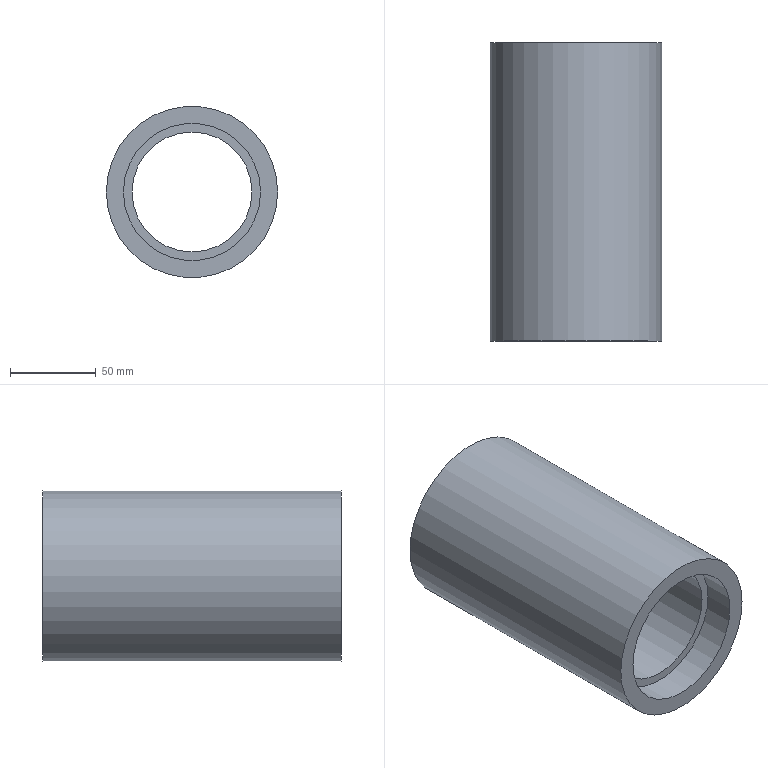Component | NX | IDLER | 1 solid | 8 faces | volume 654551 mm3 | cylinder 4 | plane 4 | commonest cylinder face diameters 80 x2 70 x1 100 x1